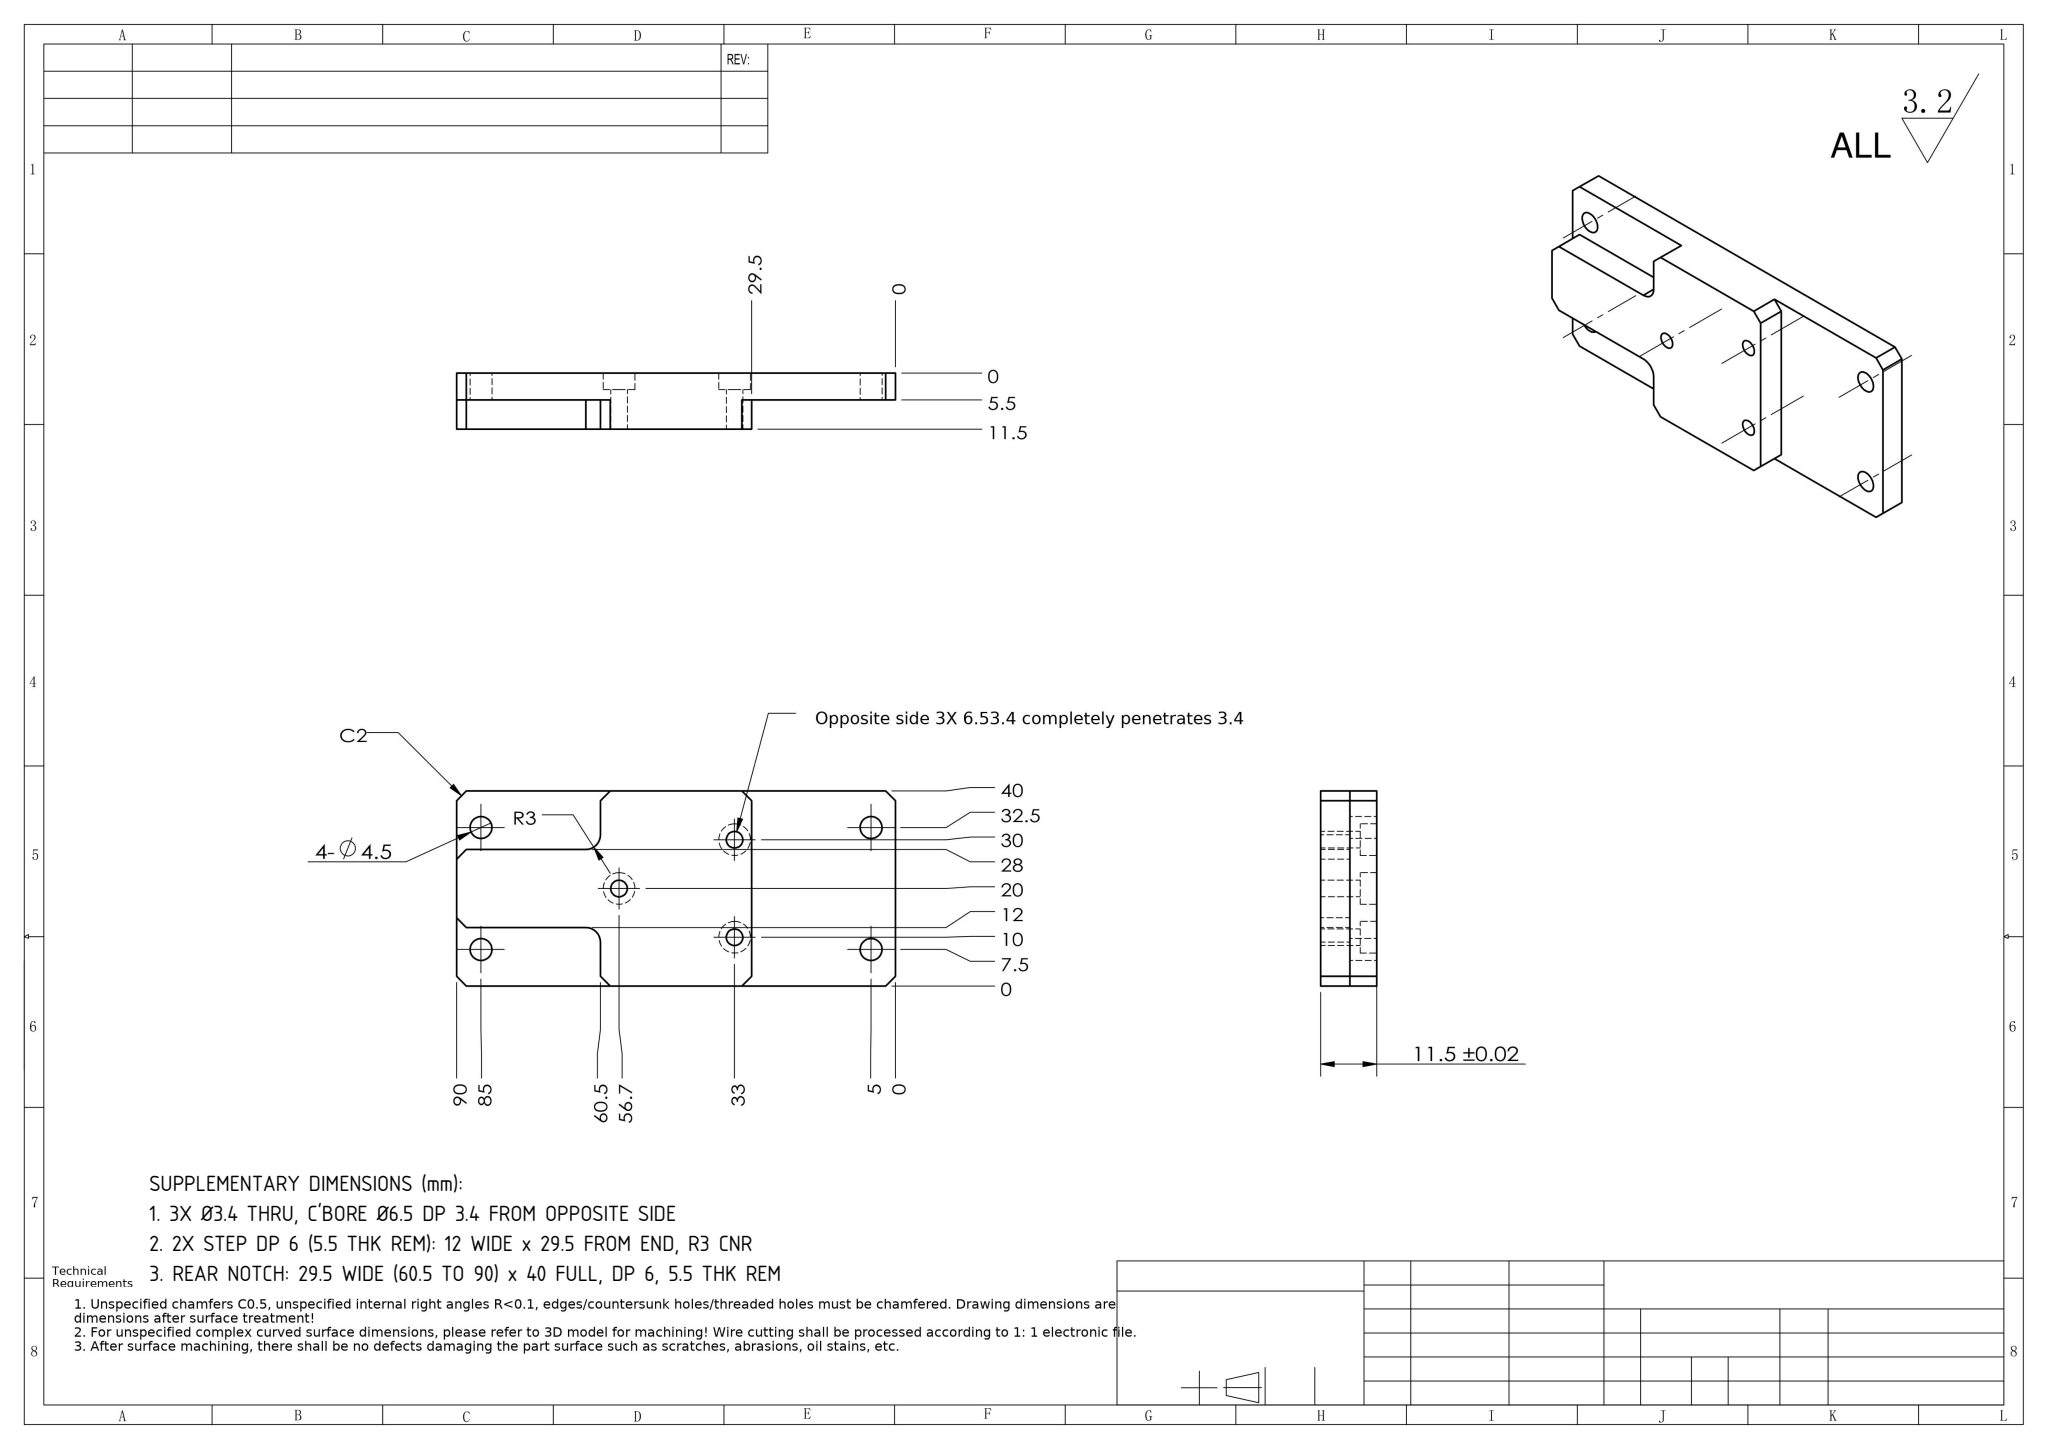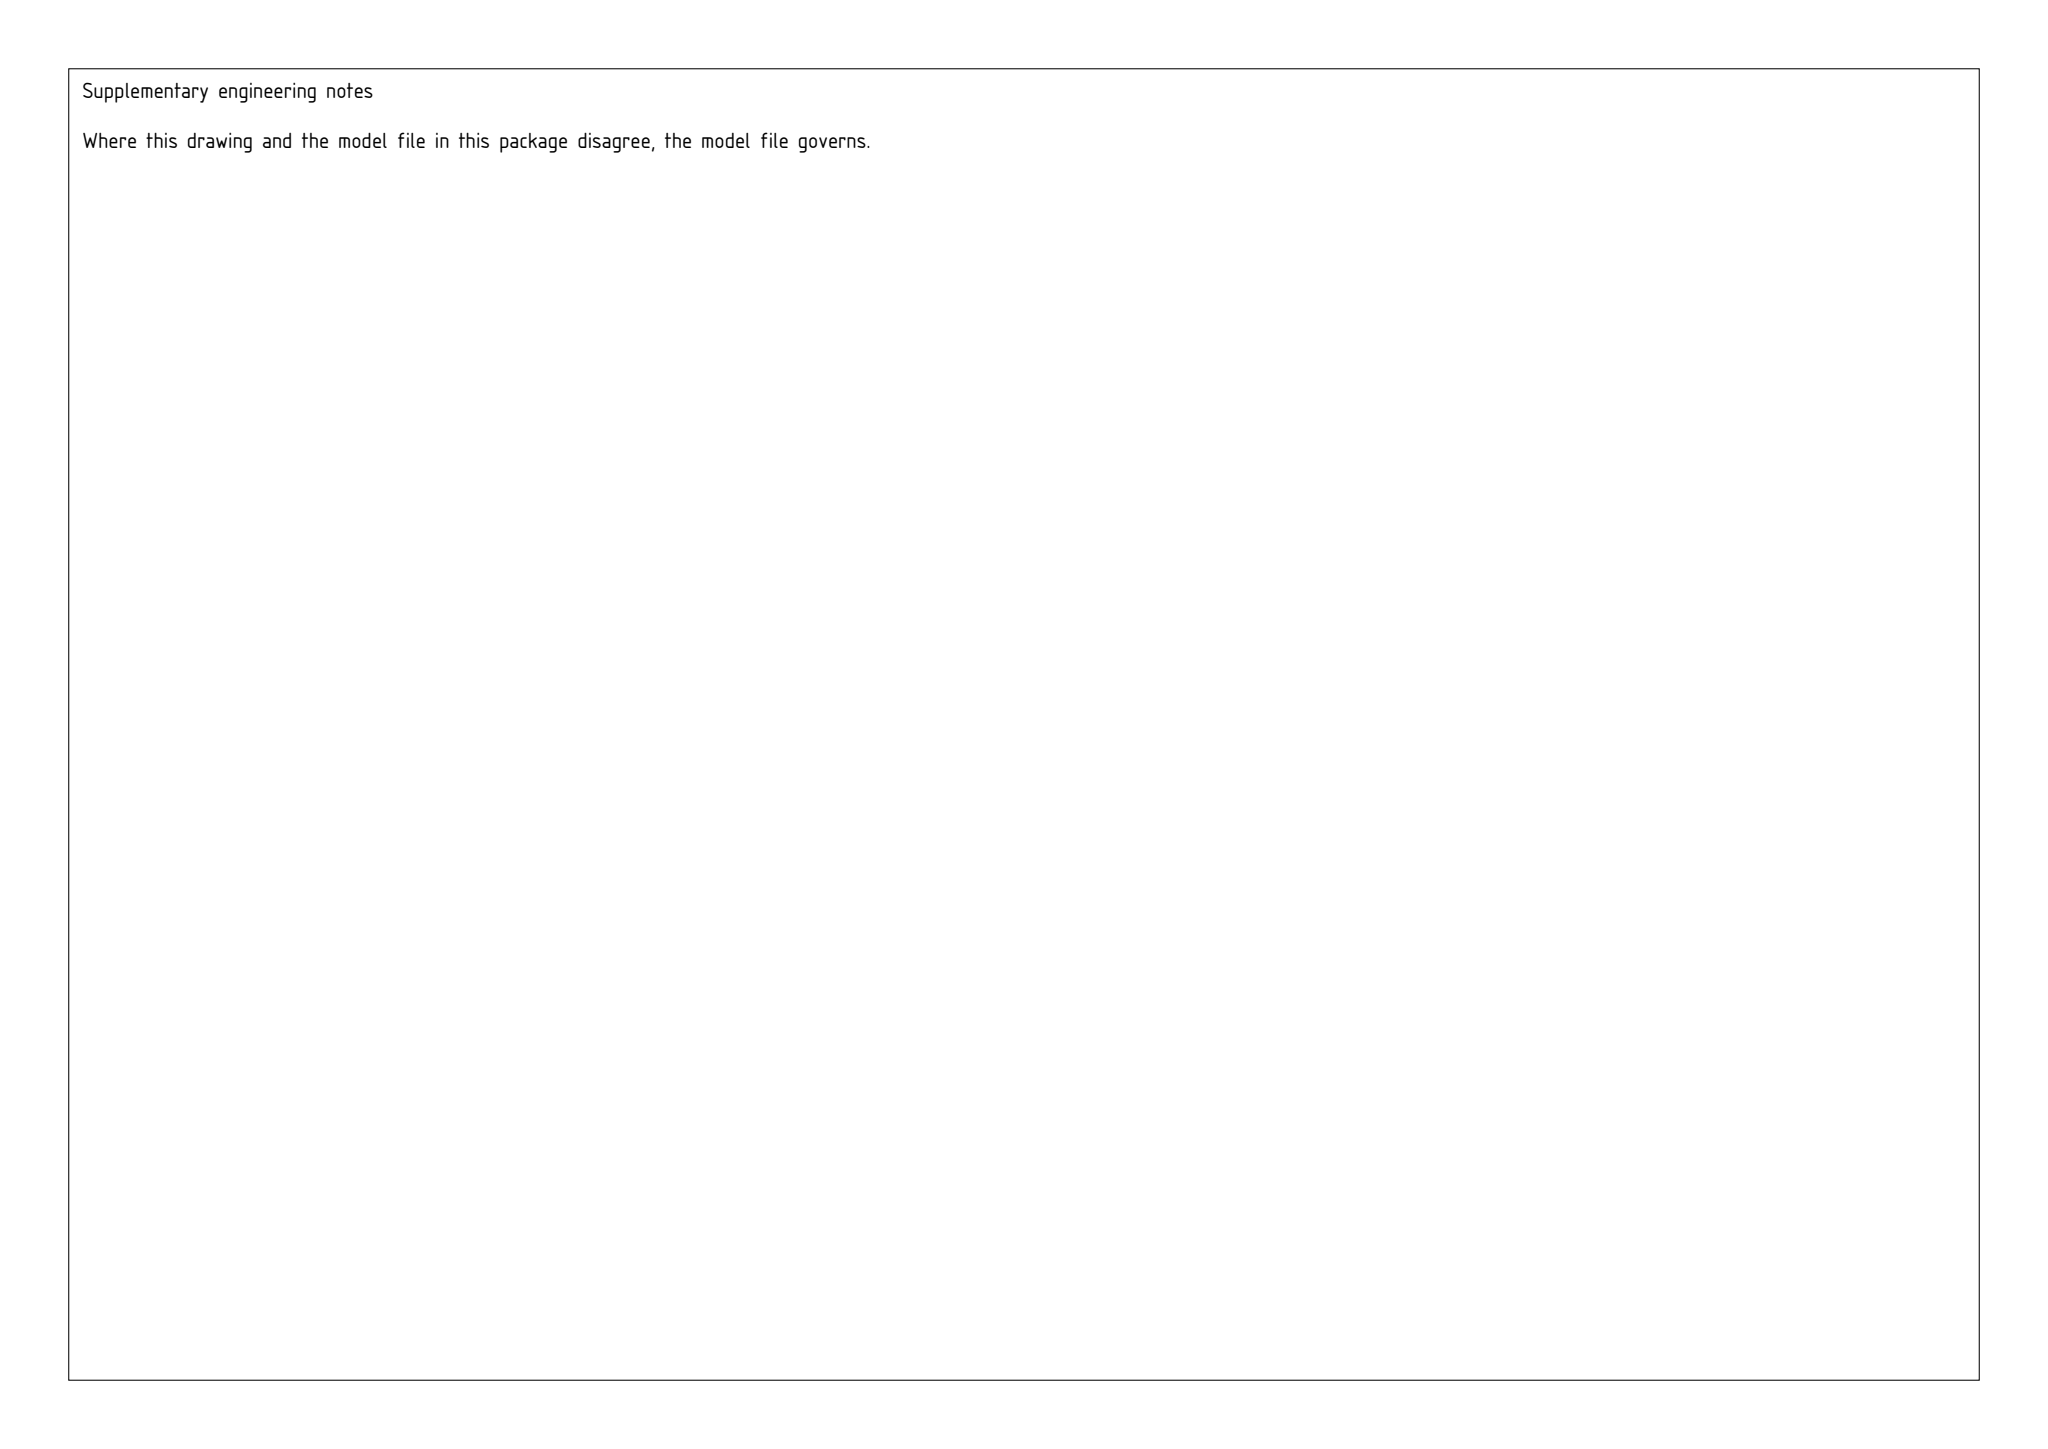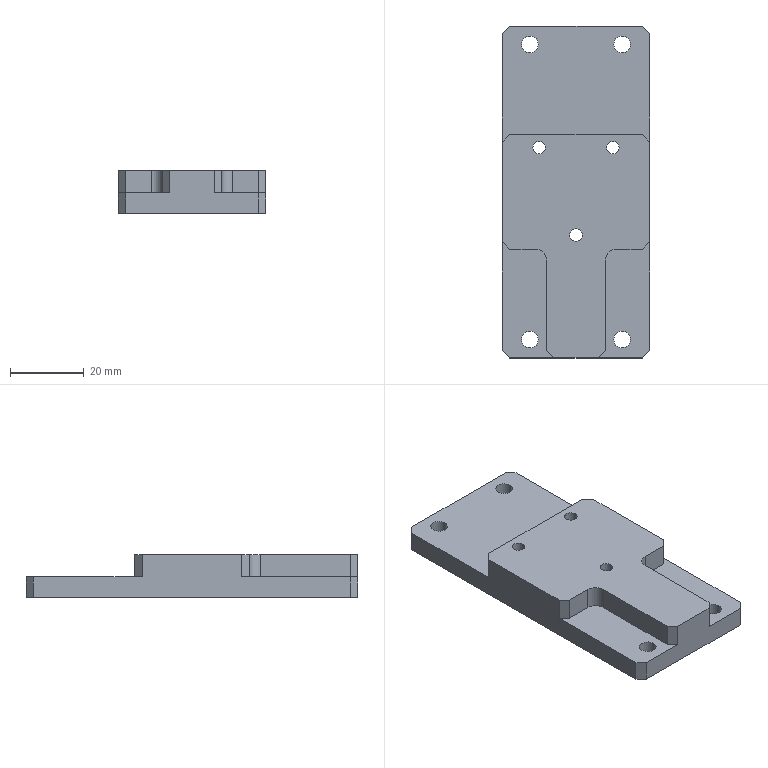Part | SolidWorks | mm | 1 solid | 49 faces | box 40 x 90 x 11.5 mm | volume 29070 mm3 | plane 27 | cylinder 22 | commonest cylinder face diameters 4.5 x8 6.5 x6 3.4 x6 6 x2
build123d program:
from build123d import *

# Parameters (mm, degrees)
SKETCH1_W                                       = 40
SKETCH1_H                                       = 90
BOSS_EXTRUDE1_DEPTH                             = 11.5
SKETCH2_W                                       = 12
SKETCH2_H                                       = 29.5
CUT_EXTRUDE1_DEPTH                              = 6
FILLET1_R                                       = 3
CHAMFER1_SIZE                                   = 2
M4_CLEARANCE_HOLE1_D                            = 4.5
CHAMFER2_SIZE                                   = 2
M3_HEX_SOCKET_HEAD_CAP_SCREW_CBORE1_D           = 3.4
M3_HEX_SOCKET_HEAD_CAP_SCREW_CBORE1_CBORE_D     = 6.5
M3_HEX_SOCKET_HEAD_CAP_SCREW_CBORE1_CBORE_DEPTH = 3.4
SKETCH8_W                                       = 30
SKETCH8_H                                       = 29.5
CUT_EXTRUDE2_DEPTH                              = 6


with BuildPart() as part:
    # Sketch1 → Boss-Extrude1 (new body)
    with BuildSketch(Plane.XY):
        Rectangle(SKETCH1_W, SKETCH1_H)
    extrude(amount=BOSS_EXTRUDE1_DEPTH)

    # Sketch2 → Cut-Extrude1 (cut)
    with BuildSketch(Plane.XY.offset(11.5)):
        with Locations((-14, 30.25)):
            Rectangle(SKETCH2_W, SKETCH2_H)
        with Locations((14, 30.25)):
            Rectangle(SKETCH2_W, SKETCH2_H)
        with Locations((14, -30.25)):
            Rectangle(SKETCH2_W, SKETCH2_H)
        with Locations((-14, -30.25)):
            Rectangle(SKETCH2_W, SKETCH2_H)
    extrude(amount=-CUT_EXTRUDE1_DEPTH, mode=Mode.SUBTRACT)

    # Fillet1
    fillet1_edges = [part.edges().sort_by_distance(p)[0] for p in [
        (-8, 15.5, 8.5),
        (8, 15.5, 8.5),
        (8, -15.5, 8.5),
        (-8, -15.5, 8.5),
    ]]
    fillet(fillet1_edges, radius=FILLET1_R)

    # Chamfer1
    chamfer1_edges = [part.edges().sort_by_distance(p)[0] for p in [
        (-20, 15.5, 8.5),
        (-8, 45, 8.5),
        (20, 15.5, 8.5),
        (8, 45, 8.5),
        (20, -15.5, 8.5),
        (8, -45, 8.5),
        (-20, -15.5, 8.5),
        (-8, -45, 8.5),
    ]]
    chamfer(chamfer1_edges, length=CHAMFER1_SIZE)

    # M4 Clearance Hole1 (through all)
    with Locations(Plane(origin=(0, 0, 0), x_dir=(-1, 0, 0), z_dir=(0, 0, -1))):
        with Locations((-12.5, 40), (12.5, 40), (-12.5, -40), (12.5, -40)):
            Hole(M4_CLEARANCE_HOLE1_D / 2)

    # Chamfer2
    chamfer2_edges = [part.edges().sort_by_distance(p)[0] for p in [
        (-20, 45, 2.75),
        (20, -45, 2.75),
        (-20, -45, 2.75),
        (20, 45, 2.75),
    ]]
    chamfer(chamfer2_edges, length=CHAMFER2_SIZE)

    # M3 Hex Socket Head Cap Screw CBORE1 (through all)
    with Locations(Plane(origin=(0, 0, 0), x_dir=(-1, 0, 0), z_dir=(0, 0, -1))):
        with Locations((10, 12), (-10, 12), (0, -11.7)):
            CounterBoreHole(M3_HEX_SOCKET_HEAD_CAP_SCREW_CBORE1_D / 2, M3_HEX_SOCKET_HEAD_CAP_SCREW_CBORE1_CBORE_D / 2, M3_HEX_SOCKET_HEAD_CAP_SCREW_CBORE1_CBORE_DEPTH)

    # Sketch8 → Cut-Extrude2 (cut)
    with BuildSketch(Plane.XY.offset(11.5)):
        with Locations((0, 30.25)):
            Rectangle(SKETCH8_W, SKETCH8_H)
    extrude(amount=-CUT_EXTRUDE2_DEPTH, mode=Mode.SUBTRACT)


solid = part.part